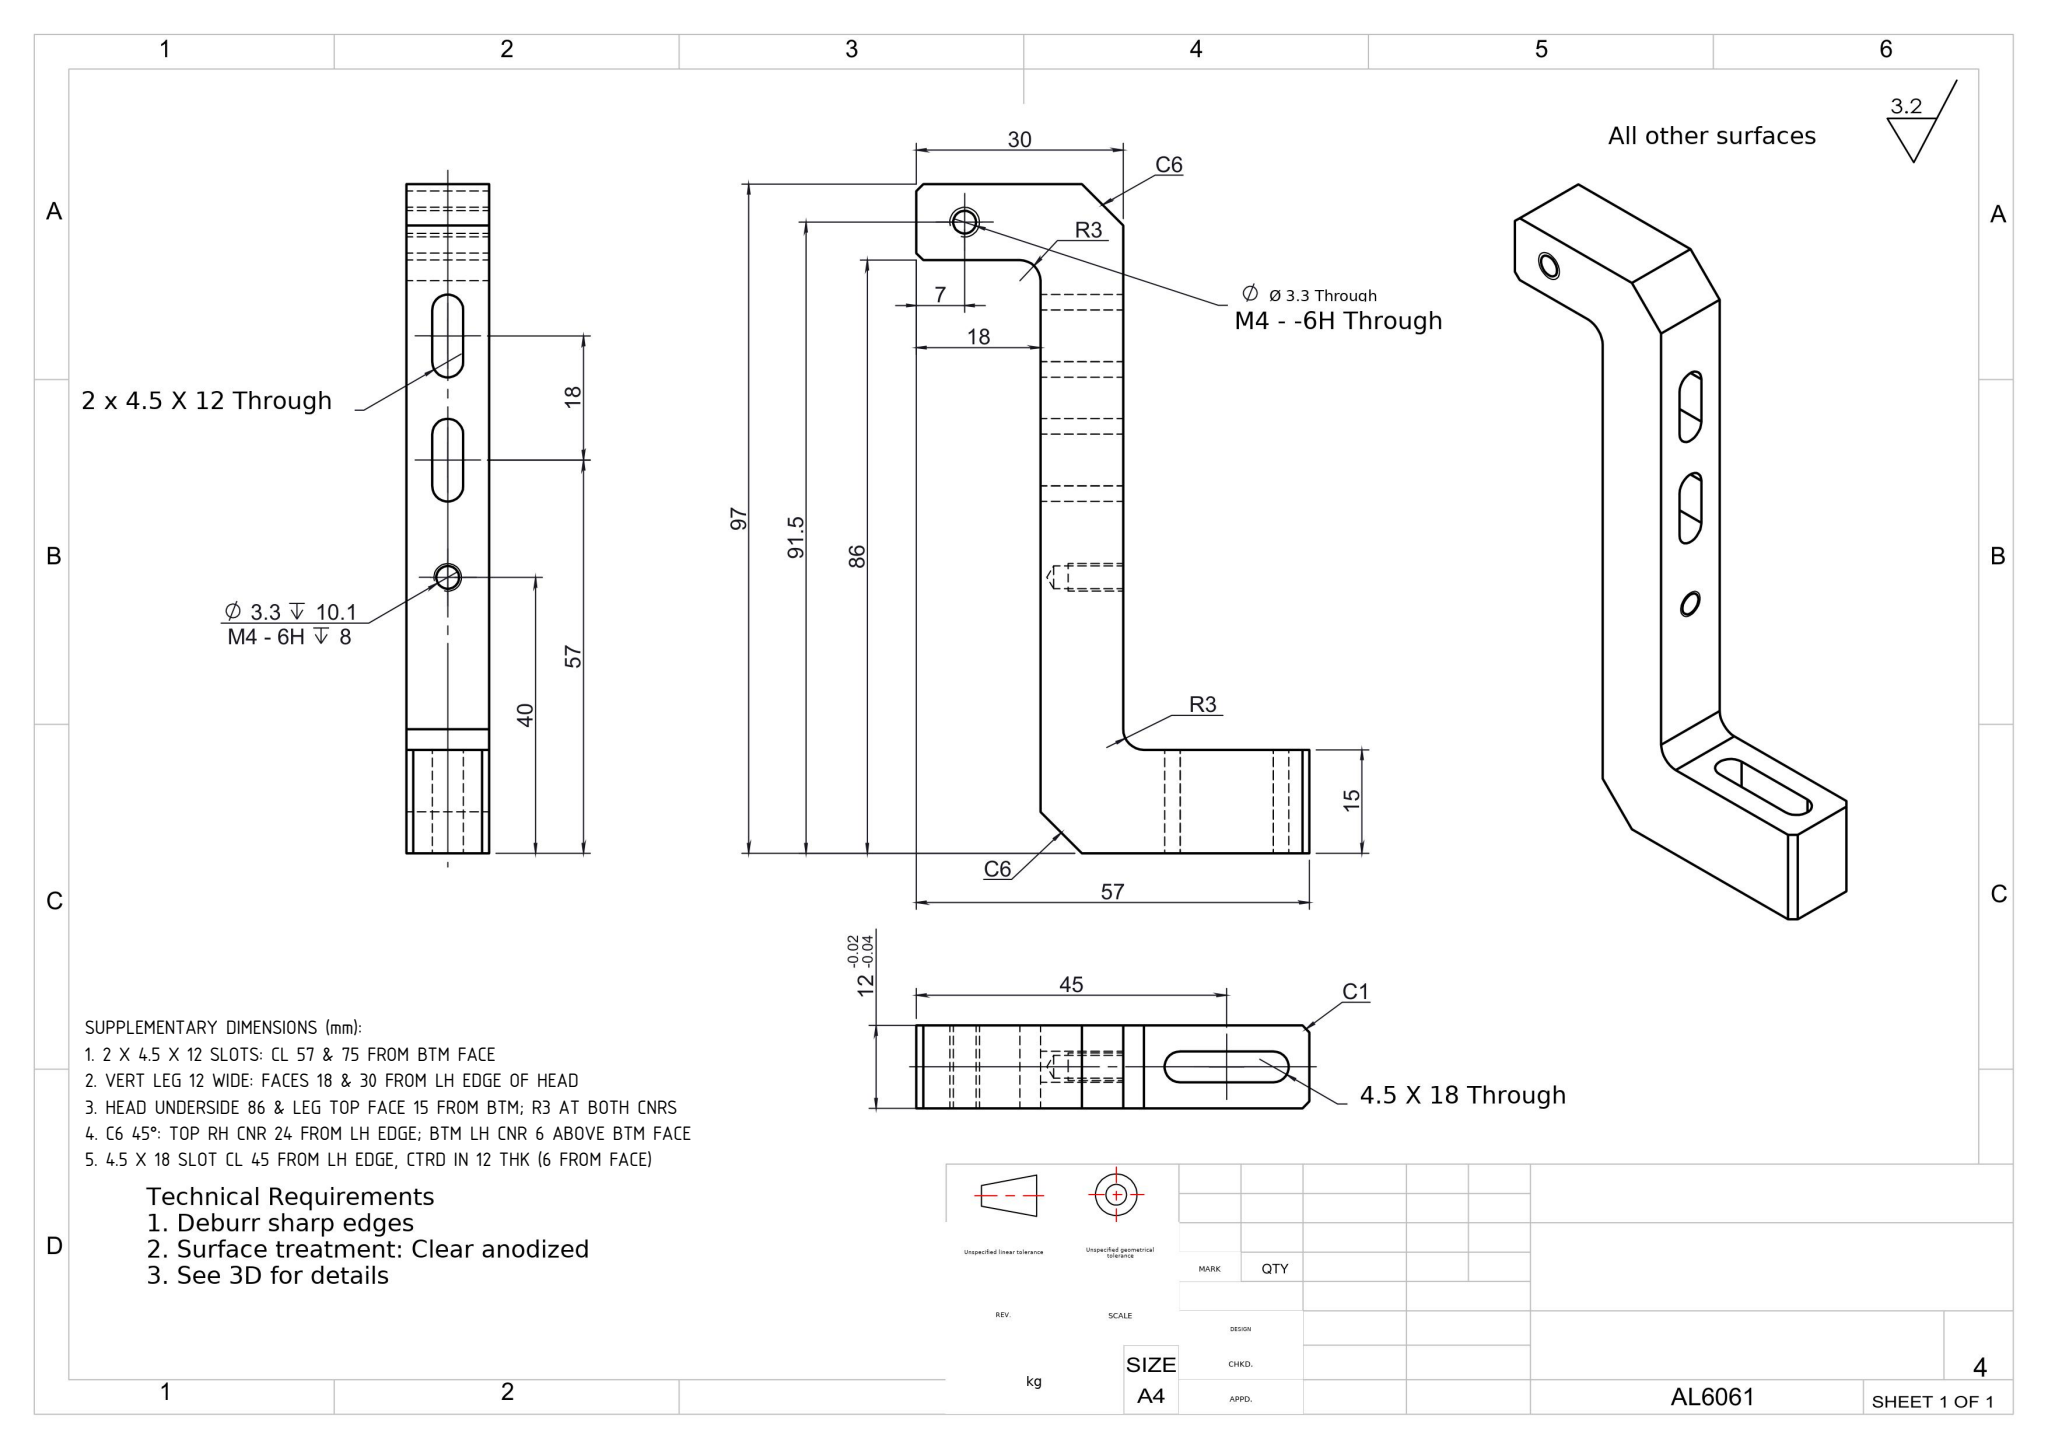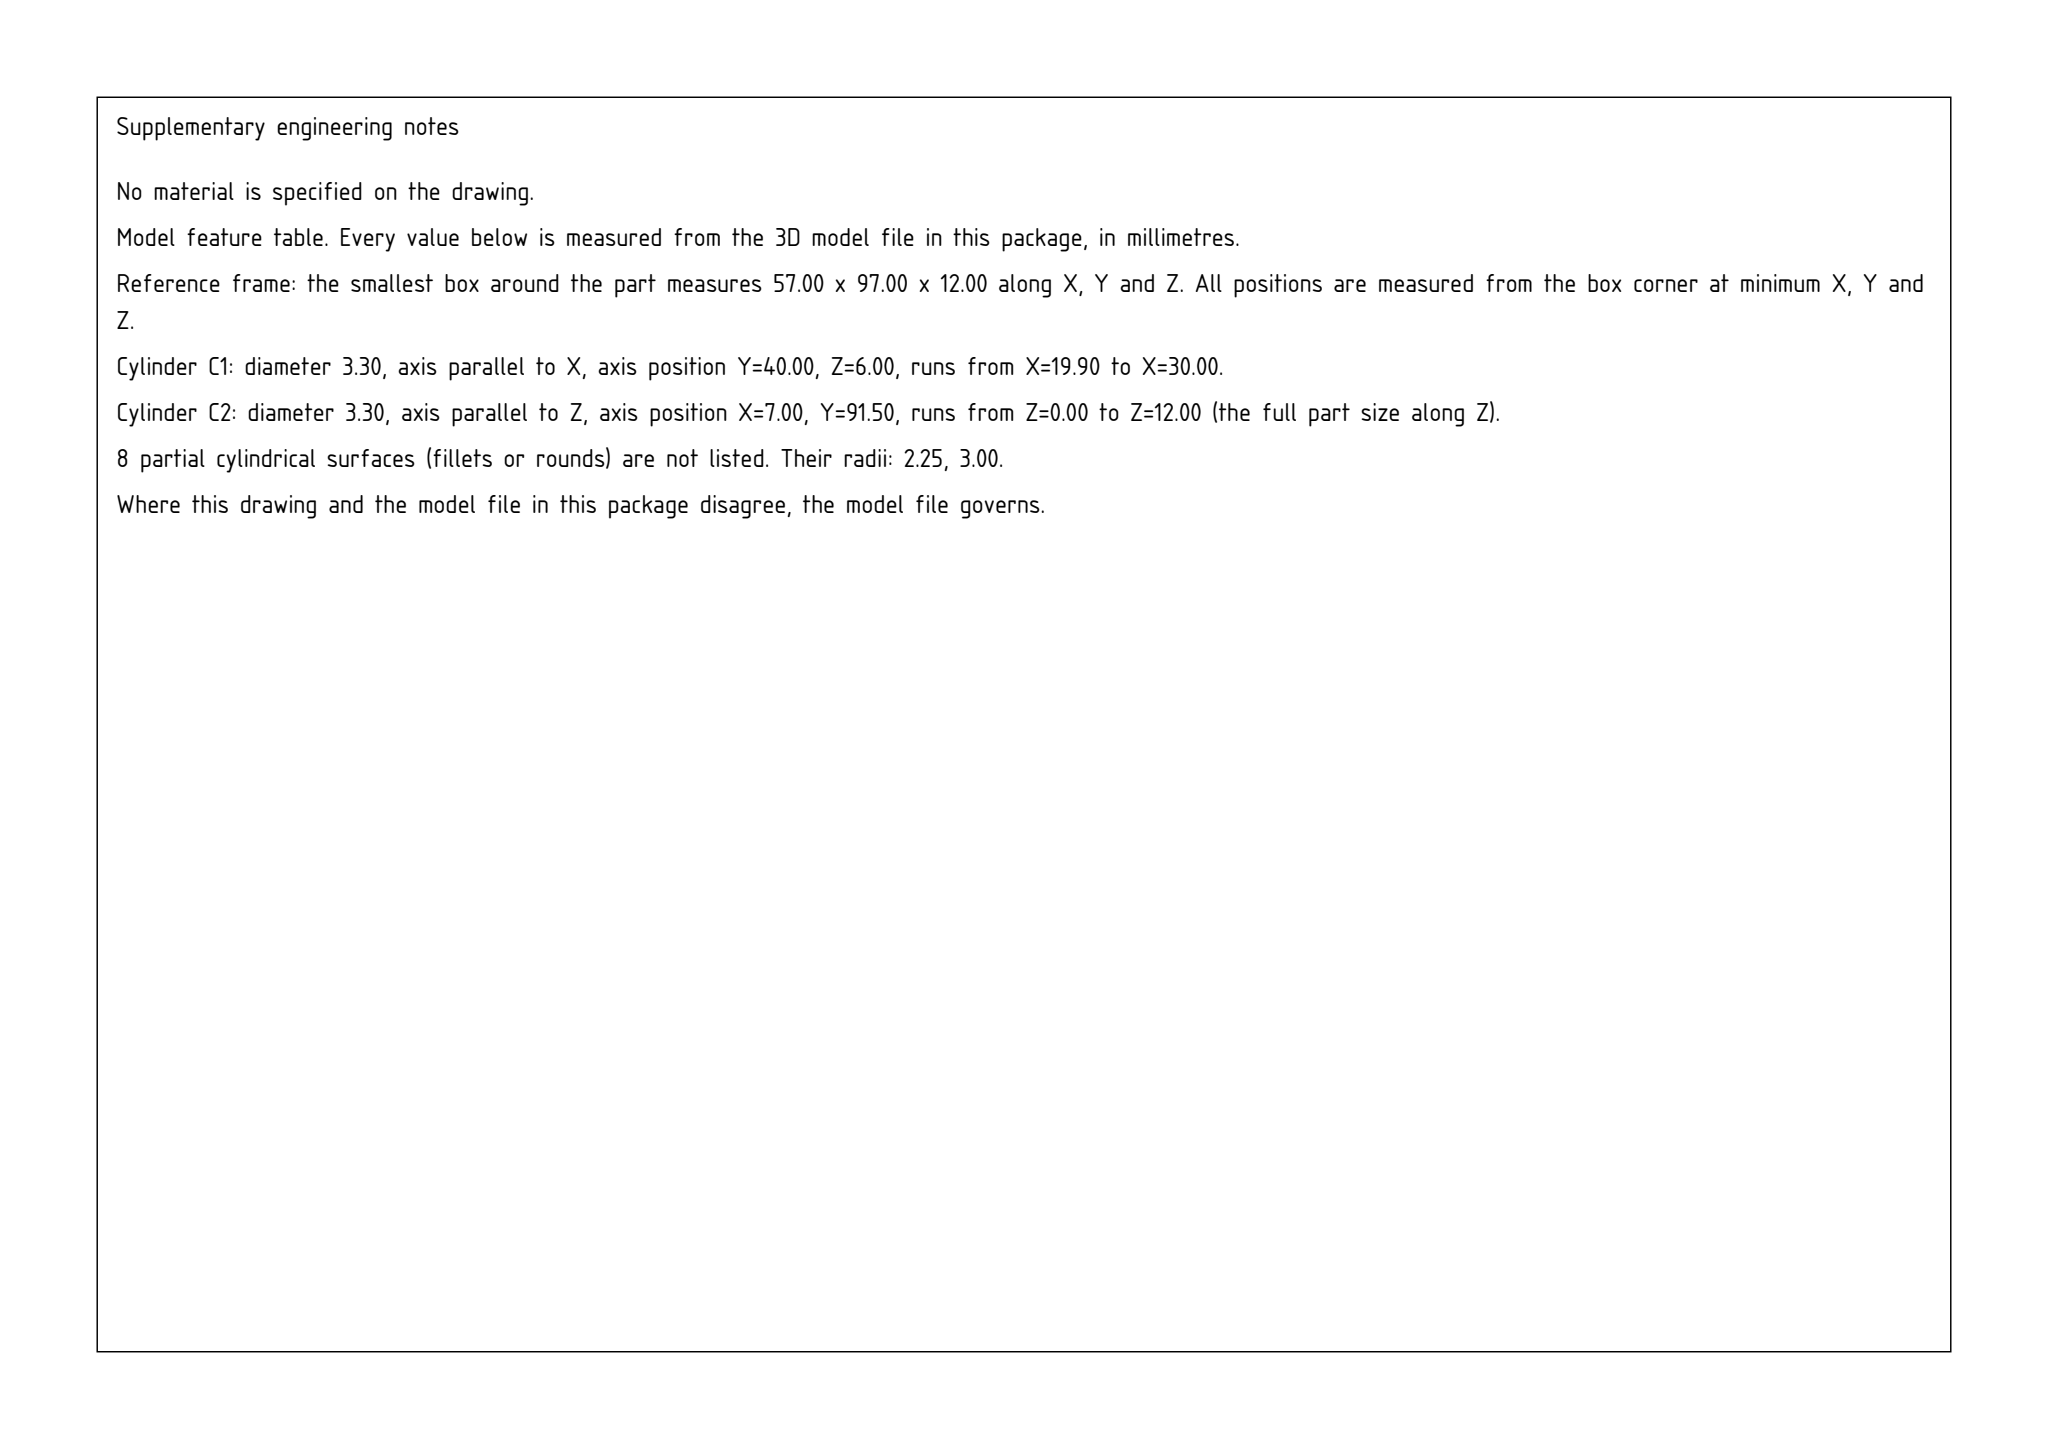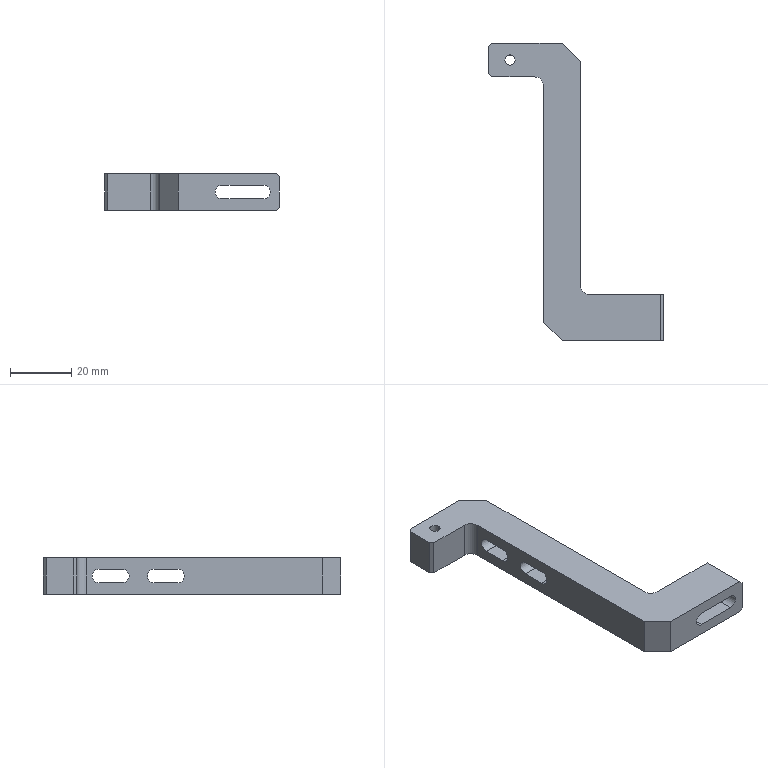Part | SolidWorks | mm | 1 solid | 36 faces | box 57 x 97 x 12 mm | volume 18258 mm3 | plane 22 | cylinder 12 | cone 2 | commonest cylinder face diameters 4.5 x6 3.3 x4 6 x2